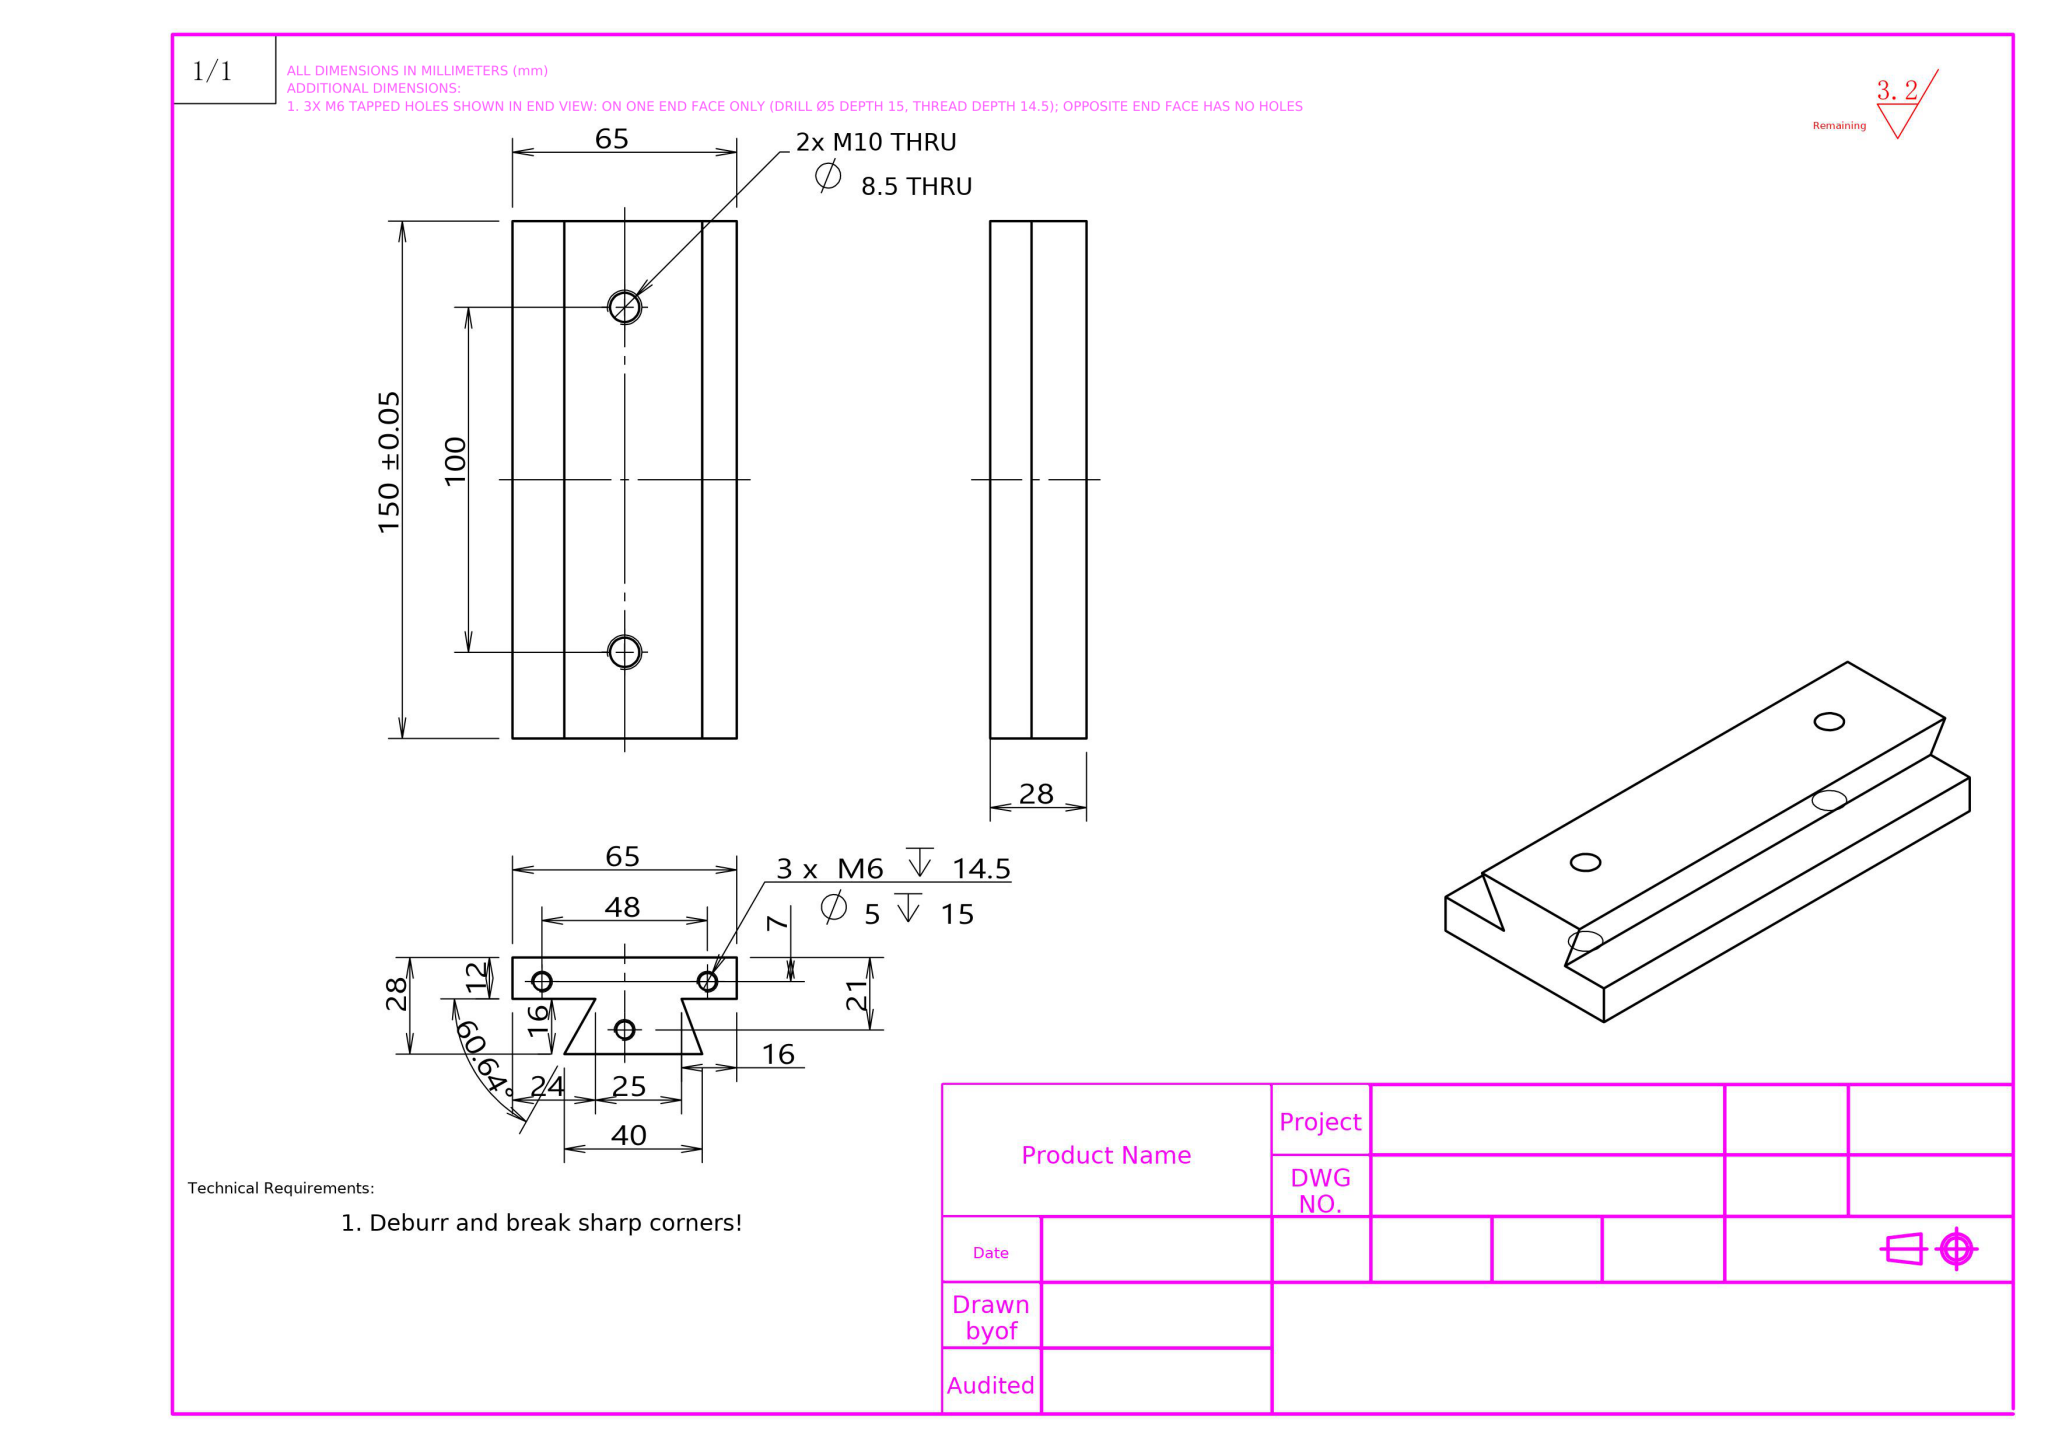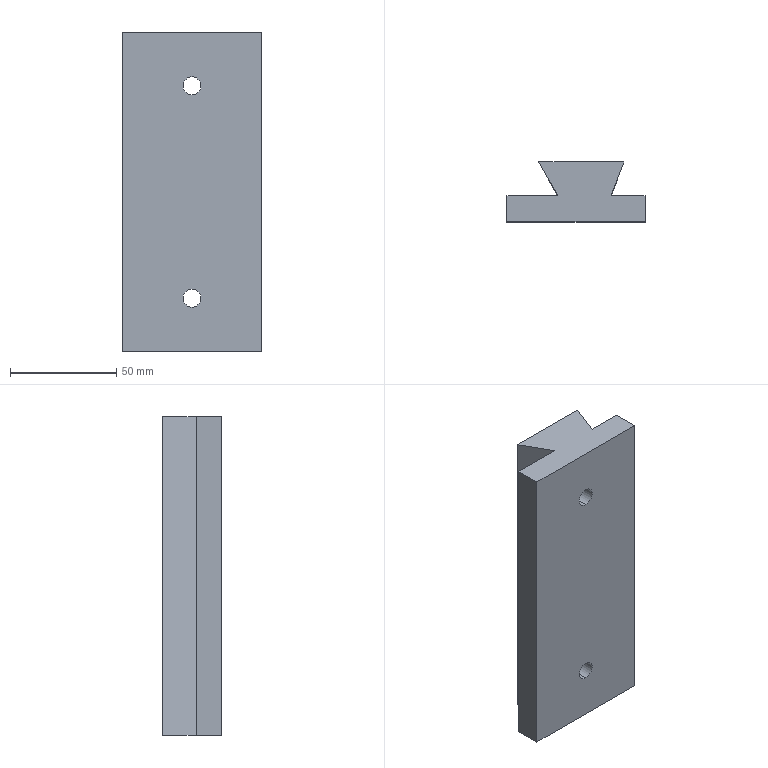Part | NX | mm | 1 solid | 26 faces | box 65 x 28 x 150 mm | volume 190909 mm3 | cylinder 10 | plane 10 | cone 6 | commonest cylinder face diameters 5 x6 8.5 x4
STEP:
#1=COLOUR_RGB('',0.7529,0.7529,0.7529);
#2=FILL_AREA_STYLE_COLOUR('',#1);
#3=FILL_AREA_STYLE('',(#2));
#4=SURFACE_STYLE_FILL_AREA(#3);
#5=SURFACE_SIDE_STYLE('',(#4));
#6=SURFACE_STYLE_USAGE(.BOTH.,#5);
#7=PRESENTATION_STYLE_ASSIGNMENT((#6));
#8=CARTESIAN_POINT('',(-21.5,1.,15.));
#9=VERTEX_POINT('',#8);
#10=CARTESIAN_POINT('',(-21.5,1.,-0.));
#11=VERTEX_POINT('',#10);
#12=CARTESIAN_POINT('',(-21.5,1.,0.));
#13=DIRECTION('',(0.,0.,-1.));
#14=VECTOR('',#13,1000.);
#15=LINE('',#12,#14);
#16=EDGE_CURVE('',#9,#11,#15,.T.);
#17=ORIENTED_EDGE('',*,*,#16,.F.);
#18=CARTESIAN_POINT('',(-26.5,1.,15.));
#19=VERTEX_POINT('',#18);
#20=CARTESIAN_POINT('',(-24.,1.,15.));
#21=DIRECTION('',(0.,0.,-1.));
#22=DIRECTION('',(-1.,0.,0.));
#23=AXIS2_PLACEMENT_3D('',#20,#21,#22);
#24=CIRCLE('',#23,2.5);
#25=EDGE_CURVE('',#19,#9,#24,.T.);
#26=ORIENTED_EDGE('',*,*,#25,.F.);
#27=CARTESIAN_POINT('',(-26.5,1.,-0.));
#28=VERTEX_POINT('',#27);
#29=CARTESIAN_POINT('',(-26.5,1.,0.));
#30=DIRECTION('',(0.,0.,-1.));
#31=VECTOR('',#30,1000.);
#32=LINE('',#29,#31);
#33=EDGE_CURVE('',#19,#28,#32,.T.);
#34=ORIENTED_EDGE('',*,*,#33,.T.);
#35=CARTESIAN_POINT('',(-24.,1.,-0.));
#36=DIRECTION('',(0.,0.,-1.));
#37=DIRECTION('',(-1.,0.,0.));
#38=AXIS2_PLACEMENT_3D('',#35,#36,#37);
#39=CIRCLE('',#38,2.5);
#40=EDGE_CURVE('',#28,#11,#39,.T.);
#41=ORIENTED_EDGE('',*,*,#40,.T.);
#42=EDGE_LOOP('',(#17,#26,#34,#41));
#43=FACE_OUTER_BOUND('',#42,.T.);
#44=CARTESIAN_POINT('',(-24.,1.,0.));
#45=DIRECTION('',(0.,0.,-1.));
#46=DIRECTION('',(-1.,0.,0.));
#47=AXIS2_PLACEMENT_3D('',#44,#45,#46);
#48=CYLINDRICAL_SURFACE('',#47,2.5);
#49=ADVANCED_FACE('',(#43),#48,.F.);
#50=STYLED_ITEM('',(#7),#49);
#51=(LENGTH_UNIT()NAMED_UNIT(*)SI_UNIT(.MILLI.,.METRE.));
#52=UNCERTAINTY_MEASURE_WITH_UNIT(LENGTH_MEASURE(0.00001),#51,'','');
#53=(NAMED_UNIT(*)PLANE_ANGLE_UNIT()SI_UNIT($,.RADIAN.));
#54=(NAMED_UNIT(*)SI_UNIT($,.STERADIAN.)SOLID_ANGLE_UNIT());
#55=(GEOMETRIC_REPRESENTATION_CONTEXT(3)GLOBAL_UNCERTAINTY_ASSIGNED_CONTEXT((#52))GLOBAL_UNIT_ASSIGNED_CONTEXT((#51,#53,#54))REPRESENTATION_CONTEXT('',''));
#56=MECHANICAL_DESIGN_GEOMETRIC_PRESENTATION_REPRESENTATION('',(#50),#55);
#57=COLOUR_RGB('',0.7529,0.7529,0.7529);
#58=FILL_AREA_STYLE_COLOUR('',#57);
#59=FILL_AREA_STYLE('',(#58));
#60=SURFACE_STYLE_FILL_AREA(#59);
#61=SURFACE_SIDE_STYLE('',(#60));
#62=SURFACE_STYLE_USAGE(.BOTH.,#61);
#63=PRESENTATION_STYLE_ASSIGNMENT((#62));
#64=CARTESIAN_POINT('',(-24.,1.,15.));
#65=DIRECTION('',(0.,0.,-1.));
#66=DIRECTION('',(-1.,0.,0.));
#67=AXIS2_PLACEMENT_3D('',#64,#65,#66);
#68=CIRCLE('',#67,2.5);
#69=EDGE_CURVE('',#9,#19,#68,.T.);
#70=ORIENTED_EDGE('',*,*,#69,.F.);
#71=ORIENTED_EDGE('',*,*,#16,.T.);
#72=CARTESIAN_POINT('',(-24.,1.,-0.));
#73=DIRECTION('',(0.,0.,-1.));
#74=DIRECTION('',(-1.,0.,0.));
#75=AXIS2_PLACEMENT_3D('',#72,#73,#74);
#76=CIRCLE('',#75,2.5);
#77=EDGE_CURVE('',#11,#28,#76,.T.);
#78=ORIENTED_EDGE('',*,*,#77,.T.);
#79=ORIENTED_EDGE('',*,*,#33,.F.);
#80=EDGE_LOOP('',(#70,#71,#78,#79));
#81=FACE_OUTER_BOUND('',#80,.T.);
#82=CARTESIAN_POINT('',(-24.,1.,0.));
#83=DIRECTION('',(0.,0.,-1.));
#84=DIRECTION('',(-1.,0.,0.));
#85=AXIS2_PLACEMENT_3D('',#82,#83,#84);
#86=CYLINDRICAL_SURFACE('',#85,2.5);
#87=ADVANCED_FACE('',(#81),#86,.F.);
#88=CARTESIAN_POINT('',(-24.,1.,16.502));
#89=VERTEX_POINT('',#88);
#90=CARTESIAN_POINT('',(-26.5,1.,15.));
#91=DIRECTION('',(-0.8572,0.,-0.515));
#92=VECTOR('',#91,1000.);
#93=LINE('',#90,#92);
#94=EDGE_CURVE('',#89,#19,#93,.T.);
#95=ORIENTED_EDGE('',*,*,#94,.F.);
#96=CARTESIAN_POINT('',(-21.5,1.,15.));
#97=DIRECTION('',(0.8572,0.,-0.515));
#98=VECTOR('',#97,1000.);
#99=LINE('',#96,#98);
#100=EDGE_CURVE('',#89,#9,#99,.T.);
#101=ORIENTED_EDGE('',*,*,#100,.T.);
#102=ORIENTED_EDGE('',*,*,#69,.T.);
#103=EDGE_LOOP('',(#95,#101,#102));
#104=FACE_OUTER_BOUND('',#103,.T.);
#105=CARTESIAN_POINT('',(-24.,1.,15.));
#106=DIRECTION('',(0.,0.,-1.));
#107=DIRECTION('',(-1.,0.,0.));
#108=AXIS2_PLACEMENT_3D('',#105,#106,#107);
#109=CONICAL_SURFACE('',#108,2.5,1.03);
#110=ADVANCED_FACE('',(#104),#109,.F.);
#111=CARTESIAN_POINT('',(2.5,15.,15.));
#112=VERTEX_POINT('',#111);
#113=CARTESIAN_POINT('',(-2.5,15.,15.));
#114=VERTEX_POINT('',#113);
#115=CARTESIAN_POINT('',(0.,15.,15.));
#116=DIRECTION('',(0.,0.,-1.));
#117=DIRECTION('',(-1.,0.,0.));
#118=AXIS2_PLACEMENT_3D('',#115,#116,#117);
#119=CIRCLE('',#118,2.5);
#120=EDGE_CURVE('',#112,#114,#119,.T.);
#121=ORIENTED_EDGE('',*,*,#120,.F.);
#122=CARTESIAN_POINT('',(2.5,15.,-0.));
#123=VERTEX_POINT('',#122);
#124=CARTESIAN_POINT('',(2.5,15.,0.));
#125=DIRECTION('',(0.,0.,-1.));
#126=VECTOR('',#125,1000.);
#127=LINE('',#124,#126);
#128=EDGE_CURVE('',#112,#123,#127,.T.);
#129=ORIENTED_EDGE('',*,*,#128,.T.);
#130=CARTESIAN_POINT('',(-2.5,15.,-0.));
#131=VERTEX_POINT('',#130);
#132=CARTESIAN_POINT('',(0.,15.,-0.));
#133=DIRECTION('',(0.,0.,-1.));
#134=DIRECTION('',(-1.,0.,0.));
#135=AXIS2_PLACEMENT_3D('',#132,#133,#134);
#136=CIRCLE('',#135,2.5);
#137=EDGE_CURVE('',#123,#131,#136,.T.);
#138=ORIENTED_EDGE('',*,*,#137,.T.);
#139=CARTESIAN_POINT('',(-2.5,15.,0.));
#140=DIRECTION('',(0.,0.,-1.));
#141=VECTOR('',#140,1000.);
#142=LINE('',#139,#141);
#143=EDGE_CURVE('',#114,#131,#142,.T.);
#144=ORIENTED_EDGE('',*,*,#143,.F.);
#145=EDGE_LOOP('',(#121,#129,#138,#144));
#146=FACE_OUTER_BOUND('',#145,.T.);
#147=CARTESIAN_POINT('',(0.,15.,0.));
#148=DIRECTION('',(0.,0.,-1.));
#149=DIRECTION('',(-1.,0.,0.));
#150=AXIS2_PLACEMENT_3D('',#147,#148,#149);
#151=CYLINDRICAL_SURFACE('',#150,2.5);
#152=ADVANCED_FACE('',(#146),#151,.F.);
#153=CARTESIAN_POINT('',(0.,15.,16.502));
#154=VERTEX_POINT('',#153);
#155=CARTESIAN_POINT('',(-2.5,15.,15.));
#156=DIRECTION('',(-0.8572,0.,-0.515));
#157=VECTOR('',#156,1000.);
#158=LINE('',#155,#157);
#159=EDGE_CURVE('',#154,#114,#158,.T.);
#160=ORIENTED_EDGE('',*,*,#159,.F.);
#161=CARTESIAN_POINT('',(2.5,15.,15.));
#162=DIRECTION('',(0.8572,0.,-0.515));
#163=VECTOR('',#162,1000.);
#164=LINE('',#161,#163);
#165=EDGE_CURVE('',#154,#112,#164,.T.);
#166=ORIENTED_EDGE('',*,*,#165,.T.);
#167=ORIENTED_EDGE('',*,*,#120,.T.);
#168=EDGE_LOOP('',(#160,#166,#167));
#169=FACE_OUTER_BOUND('',#168,.T.);
#170=CARTESIAN_POINT('',(0.,15.,15.));
#171=DIRECTION('',(0.,0.,-1.));
#172=DIRECTION('',(-1.,0.,0.));
#173=AXIS2_PLACEMENT_3D('',#170,#171,#172);
#174=CONICAL_SURFACE('',#173,2.5,1.03);
#175=ADVANCED_FACE('',(#169),#174,.F.);
#176=CARTESIAN_POINT('',(26.5,1.,15.));
#177=VERTEX_POINT('',#176);
#178=CARTESIAN_POINT('',(21.5,1.,15.));
#179=VERTEX_POINT('',#178);
#180=CARTESIAN_POINT('',(24.,1.,15.));
#181=DIRECTION('',(0.,0.,-1.));
#182=DIRECTION('',(-1.,0.,0.));
#183=AXIS2_PLACEMENT_3D('',#180,#181,#182);
#184=CIRCLE('',#183,2.5);
#185=EDGE_CURVE('',#177,#179,#184,.T.);
#186=ORIENTED_EDGE('',*,*,#185,.F.);
#187=CARTESIAN_POINT('',(26.5,1.,-0.));
#188=VERTEX_POINT('',#187);
#189=CARTESIAN_POINT('',(26.5,1.,0.));
#190=DIRECTION('',(0.,0.,-1.));
#191=VECTOR('',#190,1000.);
#192=LINE('',#189,#191);
#193=EDGE_CURVE('',#177,#188,#192,.T.);
#194=ORIENTED_EDGE('',*,*,#193,.T.);
#195=CARTESIAN_POINT('',(21.5,1.,-0.));
#196=VERTEX_POINT('',#195);
#197=CARTESIAN_POINT('',(24.,1.,-0.));
#198=DIRECTION('',(0.,0.,-1.));
#199=DIRECTION('',(-1.,0.,0.));
#200=AXIS2_PLACEMENT_3D('',#197,#198,#199);
#201=CIRCLE('',#200,2.5);
#202=EDGE_CURVE('',#188,#196,#201,.T.);
#203=ORIENTED_EDGE('',*,*,#202,.T.);
#204=CARTESIAN_POINT('',(21.5,1.,0.));
#205=DIRECTION('',(0.,0.,-1.));
#206=VECTOR('',#205,1000.);
#207=LINE('',#204,#206);
#208=EDGE_CURVE('',#179,#196,#207,.T.);
#209=ORIENTED_EDGE('',*,*,#208,.F.);
#210=EDGE_LOOP('',(#186,#194,#203,#209));
#211=FACE_OUTER_BOUND('',#210,.T.);
#212=CARTESIAN_POINT('',(24.,1.,0.));
#213=DIRECTION('',(0.,0.,-1.));
#214=DIRECTION('',(-1.,0.,0.));
#215=AXIS2_PLACEMENT_3D('',#212,#213,#214);
#216=CYLINDRICAL_SURFACE('',#215,2.5);
#217=ADVANCED_FACE('',(#211),#216,.F.);
#218=CARTESIAN_POINT('',(24.,1.,16.502));
#219=VERTEX_POINT('',#218);
#220=CARTESIAN_POINT('',(21.5,1.,15.));
#221=DIRECTION('',(-0.8572,0.,-0.515));
#222=VECTOR('',#221,1000.);
#223=LINE('',#220,#222);
#224=EDGE_CURVE('',#219,#179,#223,.T.);
#225=ORIENTED_EDGE('',*,*,#224,.F.);
#226=CARTESIAN_POINT('',(26.5,1.,15.));
#227=DIRECTION('',(0.8572,0.,-0.515));
#228=VECTOR('',#227,1000.);
#229=LINE('',#226,#228);
#230=EDGE_CURVE('',#219,#177,#229,.T.);
#231=ORIENTED_EDGE('',*,*,#230,.T.);
#232=ORIENTED_EDGE('',*,*,#185,.T.);
#233=EDGE_LOOP('',(#225,#231,#232));
#234=FACE_OUTER_BOUND('',#233,.T.);
#235=CARTESIAN_POINT('',(24.,1.,15.));
#236=DIRECTION('',(0.,0.,-1.));
#237=DIRECTION('',(-1.,0.,0.));
#238=AXIS2_PLACEMENT_3D('',#235,#236,#237);
#239=CONICAL_SURFACE('',#238,2.5,1.03);
#240=ADVANCED_FACE('',(#234),#239,.F.);
#241=CARTESIAN_POINT('',(0.,22.,129.25));
#242=VERTEX_POINT('',#241);
#243=CARTESIAN_POINT('',(0.,22.,120.75));
#244=VERTEX_POINT('',#243);
#245=CARTESIAN_POINT('',(0.,22.,125.));
#246=DIRECTION('',(0.,-1.,0.));
#247=DIRECTION('',(0.,0.,-1.));
#248=AXIS2_PLACEMENT_3D('',#245,#246,#247);
#249=CIRCLE('',#248,4.25);
#250=EDGE_CURVE('',#242,#244,#249,.T.);
#251=ORIENTED_EDGE('',*,*,#250,.F.);
#252=CARTESIAN_POINT('',(0.,-6.,129.25));
#253=VERTEX_POINT('',#252);
#254=CARTESIAN_POINT('',(0.,-6.,129.25));
#255=DIRECTION('',(0.,-1.,0.));
#256=VECTOR('',#255,1000.);
#257=LINE('',#254,#256);
#258=EDGE_CURVE('',#242,#253,#257,.T.);
#259=ORIENTED_EDGE('',*,*,#258,.T.);
#260=CARTESIAN_POINT('',(0.,-6.,120.75));
#261=VERTEX_POINT('',#260);
#262=CARTESIAN_POINT('',(0.,-6.,125.));
#263=DIRECTION('',(0.,-1.,0.));
#264=DIRECTION('',(0.,0.,-1.));
#265=AXIS2_PLACEMENT_3D('',#262,#263,#264);
#266=CIRCLE('',#265,4.25);
#267=EDGE_CURVE('',#253,#261,#266,.T.);
#268=ORIENTED_EDGE('',*,*,#267,.T.);
#269=CARTESIAN_POINT('',(0.,-6.,120.75));
#270=DIRECTION('',(0.,-1.,0.));
#271=VECTOR('',#270,1000.);
#272=LINE('',#269,#271);
#273=EDGE_CURVE('',#244,#261,#272,.T.);
#274=ORIENTED_EDGE('',*,*,#273,.F.);
#275=EDGE_LOOP('',(#251,#259,#268,#274));
#276=FACE_OUTER_BOUND('',#275,.T.);
#277=CARTESIAN_POINT('',(0.,-6.,125.));
#278=DIRECTION('',(0.,-1.,0.));
#279=DIRECTION('',(0.,0.,-1.));
#280=AXIS2_PLACEMENT_3D('',#277,#278,#279);
#281=CYLINDRICAL_SURFACE('',#280,4.25);
#282=ADVANCED_FACE('',(#276),#281,.F.);
#283=CARTESIAN_POINT('',(0.,22.,29.25));
#284=VERTEX_POINT('',#283);
#285=CARTESIAN_POINT('',(0.,22.,20.75));
#286=VERTEX_POINT('',#285);
#287=CARTESIAN_POINT('',(0.,22.,25.));
#288=DIRECTION('',(0.,-1.,0.));
#289=DIRECTION('',(0.,0.,-1.));
#290=AXIS2_PLACEMENT_3D('',#287,#288,#289);
#291=CIRCLE('',#290,4.25);
#292=EDGE_CURVE('',#284,#286,#291,.T.);
#293=ORIENTED_EDGE('',*,*,#292,.F.);
#294=CARTESIAN_POINT('',(0.,-6.,29.25));
#295=VERTEX_POINT('',#294);
#296=CARTESIAN_POINT('',(0.,-6.,29.25));
#297=DIRECTION('',(0.,-1.,0.));
#298=VECTOR('',#297,1000.);
#299=LINE('',#296,#298);
#300=EDGE_CURVE('',#284,#295,#299,.T.);
#301=ORIENTED_EDGE('',*,*,#300,.T.);
#302=CARTESIAN_POINT('',(0.,-6.,20.75));
#303=VERTEX_POINT('',#302);
#304=CARTESIAN_POINT('',(0.,-6.,25.));
#305=DIRECTION('',(0.,-1.,0.));
#306=DIRECTION('',(0.,0.,-1.));
#307=AXIS2_PLACEMENT_3D('',#304,#305,#306);
#308=CIRCLE('',#307,4.25);
#309=EDGE_CURVE('',#295,#303,#308,.T.);
#310=ORIENTED_EDGE('',*,*,#309,.T.);
#311=CARTESIAN_POINT('',(0.,-6.,20.75));
#312=DIRECTION('',(0.,-1.,0.));
#313=VECTOR('',#312,1000.);
#314=LINE('',#311,#313);
#315=EDGE_CURVE('',#286,#303,#314,.T.);
#316=ORIENTED_EDGE('',*,*,#315,.F.);
#317=EDGE_LOOP('',(#293,#301,#310,#316));
#318=FACE_OUTER_BOUND('',#317,.T.);
#319=CARTESIAN_POINT('',(0.,-6.,25.));
#320=DIRECTION('',(0.,-1.,0.));
#321=DIRECTION('',(0.,0.,-1.));
#322=AXIS2_PLACEMENT_3D('',#319,#320,#321);
#323=CYLINDRICAL_SURFACE('',#322,4.25);
#324=ADVANCED_FACE('',(#318),#323,.F.);
#325=CARTESIAN_POINT('',(32.5,-6.,0.));
#326=VERTEX_POINT('',#325);
#327=CARTESIAN_POINT('',(32.5,6.,0.));
#328=VERTEX_POINT('',#327);
#329=CARTESIAN_POINT('',(32.5,6.,0.));
#330=DIRECTION('',(0.,1.,0.));
#331=VECTOR('',#330,1000.);
#332=LINE('',#329,#331);
#333=EDGE_CURVE('',#326,#328,#332,.T.);
#334=ORIENTED_EDGE('',*,*,#333,.T.);
#335=CARTESIAN_POINT('',(32.5,6.,150.));
#336=VERTEX_POINT('',#335);
#337=CARTESIAN_POINT('',(32.5,6.,150.));
#338=DIRECTION('',(0.,0.,-1.));
#339=VECTOR('',#338,1000.);
#340=LINE('',#337,#339);
#341=EDGE_CURVE('',#336,#328,#340,.T.);
#342=ORIENTED_EDGE('',*,*,#341,.F.);
#343=CARTESIAN_POINT('',(32.5,-6.,150.));
#344=VERTEX_POINT('',#343);
#345=CARTESIAN_POINT('',(32.5,6.,150.));
#346=DIRECTION('',(0.,1.,0.));
#347=VECTOR('',#346,1000.);
#348=LINE('',#345,#347);
#349=EDGE_CURVE('',#344,#336,#348,.T.);
#350=ORIENTED_EDGE('',*,*,#349,.F.);
#351=CARTESIAN_POINT('',(32.5,-6.,150.));
#352=DIRECTION('',(0.,0.,-1.));
#353=VECTOR('',#352,1000.);
#354=LINE('',#351,#353);
#355=EDGE_CURVE('',#344,#326,#354,.T.);
#356=ORIENTED_EDGE('',*,*,#355,.T.);
#357=EDGE_LOOP('',(#334,#342,#350,#356));
#358=FACE_OUTER_BOUND('',#357,.T.);
#359=CARTESIAN_POINT('',(32.5,6.,150.));
#360=DIRECTION('',(-1.,0.,0.));
#361=DIRECTION('',(0.,0.,1.));
#362=AXIS2_PLACEMENT_3D('',#359,#360,#361);
#363=PLANE('',#362);
#364=ADVANCED_FACE('',(#358),#363,.F.);
#365=CARTESIAN_POINT('',(16.5,6.,0.));
#366=VERTEX_POINT('',#365);
#367=CARTESIAN_POINT('',(16.5,6.,0.));
#368=DIRECTION('',(-1.,0.,0.));
#369=VECTOR('',#368,1000.);
#370=LINE('',#367,#369);
#371=EDGE_CURVE('',#328,#366,#370,.T.);
#372=ORIENTED_EDGE('',*,*,#371,.T.);
#373=CARTESIAN_POINT('',(16.5,6.,150.));
#374=VERTEX_POINT('',#373);
#375=CARTESIAN_POINT('',(16.5,6.,150.));
#376=DIRECTION('',(0.,0.,-1.));
#377=VECTOR('',#376,1000.);
#378=LINE('',#375,#377);
#379=EDGE_CURVE('',#374,#366,#378,.T.);
#380=ORIENTED_EDGE('',*,*,#379,.F.);
#381=CARTESIAN_POINT('',(16.5,6.,150.));
#382=DIRECTION('',(-1.,0.,0.));
#383=VECTOR('',#382,1000.);
#384=LINE('',#381,#383);
#385=EDGE_CURVE('',#336,#374,#384,.T.);
#386=ORIENTED_EDGE('',*,*,#385,.F.);
#387=ORIENTED_EDGE('',*,*,#341,.T.);
#388=EDGE_LOOP('',(#372,#380,#386,#387));
#389=FACE_OUTER_BOUND('',#388,.T.);
#390=CARTESIAN_POINT('',(16.5,6.,150.));
#391=DIRECTION('',(0.,-1.,0.));
#392=DIRECTION('',(0.,0.,-1.));
#393=AXIS2_PLACEMENT_3D('',#390,#391,#392);
#394=PLANE('',#393);
#395=ADVANCED_FACE('',(#389),#394,.F.);
#396=CARTESIAN_POINT('',(22.5,22.,0.));
#397=VERTEX_POINT('',#396);
#398=CARTESIAN_POINT('',(22.5,22.,0.));
#399=DIRECTION('',(0.3511,0.9363,0.));
#400=VECTOR('',#399,1000.);
#401=LINE('',#398,#400);
#402=EDGE_CURVE('',#366,#397,#401,.T.);
#403=ORIENTED_EDGE('',*,*,#402,.T.);
#404=CARTESIAN_POINT('',(22.5,22.,150.));
#405=VERTEX_POINT('',#404);
#406=CARTESIAN_POINT('',(22.5,22.,150.));
#407=DIRECTION('',(0.,0.,-1.));
#408=VECTOR('',#407,1000.);
#409=LINE('',#406,#408);
#410=EDGE_CURVE('',#405,#397,#409,.T.);
#411=ORIENTED_EDGE('',*,*,#410,.F.);
#412=CARTESIAN_POINT('',(22.5,22.,150.));
#413=DIRECTION('',(0.3511,0.9363,0.));
#414=VECTOR('',#413,1000.);
#415=LINE('',#412,#414);
#416=EDGE_CURVE('',#374,#405,#415,.T.);
#417=ORIENTED_EDGE('',*,*,#416,.F.);
#418=ORIENTED_EDGE('',*,*,#379,.T.);
#419=EDGE_LOOP('',(#403,#411,#417,#418));
#420=FACE_OUTER_BOUND('',#419,.T.);
#421=CARTESIAN_POINT('',(22.5,22.,150.));
#422=DIRECTION('',(-0.9363,0.3511,0.));
#423=DIRECTION('',(-0.3511,-0.9363,0.));
#424=AXIS2_PLACEMENT_3D('',#421,#422,#423);
#425=PLANE('',#424);
#426=ADVANCED_FACE('',(#420),#425,.F.);
#427=CARTESIAN_POINT('',(0.,22.,125.));
#428=DIRECTION('',(0.,-1.,0.));
#429=DIRECTION('',(0.,0.,-1.));
#430=AXIS2_PLACEMENT_3D('',#427,#428,#429);
#431=CIRCLE('',#430,4.25);
#432=EDGE_CURVE('',#244,#242,#431,.T.);
#433=ORIENTED_EDGE('',*,*,#432,.T.);
#434=ORIENTED_EDGE('',*,*,#250,.T.);
#435=EDGE_LOOP('',(#433,#434));
#436=FACE_BOUND('',#435,.T.);
#437=CARTESIAN_POINT('',(0.,22.,25.));
#438=DIRECTION('',(0.,-1.,0.));
#439=DIRECTION('',(0.,0.,-1.));
#440=AXIS2_PLACEMENT_3D('',#437,#438,#439);
#441=CIRCLE('',#440,4.25);
#442=EDGE_CURVE('',#286,#284,#441,.T.);
#443=ORIENTED_EDGE('',*,*,#442,.T.);
#444=ORIENTED_EDGE('',*,*,#292,.T.);
#445=EDGE_LOOP('',(#443,#444));
#446=FACE_BOUND('',#445,.T.);
#447=CARTESIAN_POINT('',(-17.5,22.,0.));
#448=VERTEX_POINT('',#447);
#449=CARTESIAN_POINT('',(-17.5,22.,0.));
#450=DIRECTION('',(-1.,0.,0.));
#451=VECTOR('',#450,1000.);
#452=LINE('',#449,#451);
#453=EDGE_CURVE('',#397,#448,#452,.T.);
#454=ORIENTED_EDGE('',*,*,#453,.T.);
#455=CARTESIAN_POINT('',(-17.5,22.,150.));
#456=VERTEX_POINT('',#455);
#457=CARTESIAN_POINT('',(-17.5,22.,150.));
#458=DIRECTION('',(0.,0.,-1.));
#459=VECTOR('',#458,1000.);
#460=LINE('',#457,#459);
#461=EDGE_CURVE('',#456,#448,#460,.T.);
#462=ORIENTED_EDGE('',*,*,#461,.F.);
#463=CARTESIAN_POINT('',(-17.5,22.,150.));
#464=DIRECTION('',(-1.,0.,0.));
#465=VECTOR('',#464,1000.);
#466=LINE('',#463,#465);
#467=EDGE_CURVE('',#405,#456,#466,.T.);
#468=ORIENTED_EDGE('',*,*,#467,.F.);
#469=ORIENTED_EDGE('',*,*,#410,.T.);
#470=EDGE_LOOP('',(#454,#462,#468,#469));
#471=FACE_OUTER_BOUND('',#470,.T.);
#472=CARTESIAN_POINT('',(-17.5,22.,150.));
#473=DIRECTION('',(0.,-1.,0.));
#474=DIRECTION('',(0.,0.,-1.));
#475=AXIS2_PLACEMENT_3D('',#472,#473,#474);
#476=PLANE('',#475);
#477=ADVANCED_FACE('',(#436,#446,#471),#476,.F.);
#478=CARTESIAN_POINT('',(-8.5,6.,0.));
#479=VERTEX_POINT('',#478);
#480=CARTESIAN_POINT('',(-8.5,6.,0.));
#481=DIRECTION('',(0.4903,-0.8716,0.));
#482=VECTOR('',#481,1000.);
#483=LINE('',#480,#482);
#484=EDGE_CURVE('',#448,#479,#483,.T.);
#485=ORIENTED_EDGE('',*,*,#484,.T.);
#486=CARTESIAN_POINT('',(-8.5,6.,150.));
#487=VERTEX_POINT('',#486);
#488=CARTESIAN_POINT('',(-8.5,6.,150.));
#489=DIRECTION('',(0.,0.,-1.));
#490=VECTOR('',#489,1000.);
#491=LINE('',#488,#490);
#492=EDGE_CURVE('',#487,#479,#491,.T.);
#493=ORIENTED_EDGE('',*,*,#492,.F.);
#494=CARTESIAN_POINT('',(-8.5,6.,150.));
#495=DIRECTION('',(0.4903,-0.8716,0.));
#496=VECTOR('',#495,1000.);
#497=LINE('',#494,#496);
#498=EDGE_CURVE('',#456,#487,#497,.T.);
#499=ORIENTED_EDGE('',*,*,#498,.F.);
#500=ORIENTED_EDGE('',*,*,#461,.T.);
#501=EDGE_LOOP('',(#485,#493,#499,#500));
#502=FACE_OUTER_BOUND('',#501,.T.);
#503=CARTESIAN_POINT('',(-8.5,6.,150.));
#504=DIRECTION('',(0.8716,0.4903,0.));
#505=DIRECTION('',(-0.4903,0.8716,0.));
#506=AXIS2_PLACEMENT_3D('',#503,#504,#505);
#507=PLANE('',#506);
#508=ADVANCED_FACE('',(#502),#507,.F.);
#509=CARTESIAN_POINT('',(-32.5,6.,0.));
#510=VERTEX_POINT('',#509);
#511=CARTESIAN_POINT('',(-32.5,6.,0.));
#512=DIRECTION('',(-1.,0.,0.));
#513=VECTOR('',#512,1000.);
#514=LINE('',#511,#513);
#515=EDGE_CURVE('',#479,#510,#514,.T.);
#516=ORIENTED_EDGE('',*,*,#515,.T.);
#517=CARTESIAN_POINT('',(-32.5,6.,150.));
#518=VERTEX_POINT('',#517);
#519=CARTESIAN_POINT('',(-32.5,6.,150.));
#520=DIRECTION('',(0.,0.,-1.));
#521=VECTOR('',#520,1000.);
#522=LINE('',#519,#521);
#523=EDGE_CURVE('',#518,#510,#522,.T.);
#524=ORIENTED_EDGE('',*,*,#523,.F.);
#525=CARTESIAN_POINT('',(-32.5,6.,150.));
#526=DIRECTION('',(-1.,0.,0.));
#527=VECTOR('',#526,1000.);
#528=LINE('',#525,#527);
#529=EDGE_CURVE('',#487,#518,#528,.T.);
#530=ORIENTED_EDGE('',*,*,#529,.F.);
#531=ORIENTED_EDGE('',*,*,#492,.T.);
#532=EDGE_LOOP('',(#516,#524,#530,#531));
#533=FACE_OUTER_BOUND('',#532,.T.);
#534=CARTESIAN_POINT('',(-32.5,6.,150.));
#535=DIRECTION('',(0.,-1.,0.));
#536=DIRECTION('',(0.,0.,-1.));
#537=AXIS2_PLACEMENT_3D('',#534,#535,#536);
#538=PLANE('',#537);
#539=ADVANCED_FACE('',(#533),#538,.F.);
#540=CARTESIAN_POINT('',(-32.5,-6.,0.));
#541=VERTEX_POINT('',#540);
#542=CARTESIAN_POINT('',(-32.5,6.,0.));
#543=DIRECTION('',(0.,-1.,0.));
#544=VECTOR('',#543,1000.);
#545=LINE('',#542,#544);
#546=EDGE_CURVE('',#510,#541,#545,.T.);
#547=ORIENTED_EDGE('',*,*,#546,.T.);
#548=CARTESIAN_POINT('',(-32.5,-6.,150.));
#549=VERTEX_POINT('',#548);
#550=CARTESIAN_POINT('',(-32.5,-6.,150.));
#551=DIRECTION('',(0.,0.,-1.));
#552=VECTOR('',#551,1000.);
#553=LINE('',#550,#552);
#554=EDGE_CURVE('',#549,#541,#553,.T.);
#555=ORIENTED_EDGE('',*,*,#554,.F.);
#556=CARTESIAN_POINT('',(-32.5,6.,150.));
#557=DIRECTION('',(0.,-1.,0.));
#558=VECTOR('',#557,1000.);
#559=LINE('',#556,#558);
#560=EDGE_CURVE('',#518,#549,#559,.T.);
#561=ORIENTED_EDGE('',*,*,#560,.F.);
#562=ORIENTED_EDGE('',*,*,#523,.T.);
#563=EDGE_LOOP('',(#547,#555,#561,#562));
#564=FACE_OUTER_BOUND('',#563,.T.);
#565=CARTESIAN_POINT('',(-32.5,6.,150.));
#566=DIRECTION('',(1.,0.,0.));
#567=DIRECTION('',(0.,0.,-1.));
#568=AXIS2_PLACEMENT_3D('',#565,#566,#567);
#569=PLANE('',#568);
#570=ADVANCED_FACE('',(#564),#569,.F.);
#571=CARTESIAN_POINT('',(0.,-6.,125.));
#572=DIRECTION('',(0.,-1.,0.));
#573=DIRECTION('',(0.,0.,-1.));
#574=AXIS2_PLACEMENT_3D('',#571,#572,#573);
#575=CIRCLE('',#574,4.25);
#576=EDGE_CURVE('',#261,#253,#575,.T.);
#577=ORIENTED_EDGE('',*,*,#576,.F.);
#578=ORIENTED_EDGE('',*,*,#267,.F.);
#579=EDGE_LOOP('',(#577,#578));
#580=FACE_BOUND('',#579,.T.);
#581=CARTESIAN_POINT('',(0.,-6.,25.));
#582=DIRECTION('',(0.,-1.,0.));
#583=DIRECTION('',(0.,0.,-1.));
#584=AXIS2_PLACEMENT_3D('',#581,#582,#583);
#585=CIRCLE('',#584,4.25);
#586=EDGE_CURVE('',#303,#295,#585,.T.);
#587=ORIENTED_EDGE('',*,*,#586,.F.);
#588=ORIENTED_EDGE('',*,*,#309,.F.);
#589=EDGE_LOOP('',(#587,#588));
#590=FACE_BOUND('',#589,.T.);
#591=CARTESIAN_POINT('',(-32.5,-6.,0.));
#592=DIRECTION('',(1.,0.,0.));
#593=VECTOR('',#592,1000.);
#594=LINE('',#591,#593);
#595=EDGE_CURVE('',#541,#326,#594,.T.);
#596=ORIENTED_EDGE('',*,*,#595,.T.);
#597=ORIENTED_EDGE('',*,*,#355,.F.);
#598=CARTESIAN_POINT('',(-32.5,-6.,150.));
#599=DIRECTION('',(1.,0.,0.));
#600=VECTOR('',#599,1000.);
#601=LINE('',#598,#600);
#602=EDGE_CURVE('',#549,#344,#601,.T.);
#603=ORIENTED_EDGE('',*,*,#602,.F.);
#604=ORIENTED_EDGE('',*,*,#554,.T.);
#605=EDGE_LOOP('',(#596,#597,#603,#604));
#606=FACE_OUTER_BOUND('',#605,.T.);
#607=CARTESIAN_POINT('',(-32.5,-6.,150.));
#608=DIRECTION('',(0.,1.,0.));
#609=DIRECTION('',(0.,0.,1.));
#610=AXIS2_PLACEMENT_3D('',#607,#608,#609);
#611=PLANE('',#610);
#612=ADVANCED_FACE('',(#580,#590,#606),#611,.F.);
#613=ORIENTED_EDGE('',*,*,#349,.T.);
#614=ORIENTED_EDGE('',*,*,#385,.T.);
#615=ORIENTED_EDGE('',*,*,#416,.T.);
#616=ORIENTED_EDGE('',*,*,#467,.T.);
#617=ORIENTED_EDGE('',*,*,#498,.T.);
#618=ORIENTED_EDGE('',*,*,#529,.T.);
#619=ORIENTED_EDGE('',*,*,#560,.T.);
#620=ORIENTED_EDGE('',*,*,#602,.T.);
#621=EDGE_LOOP('',(#613,#614,#615,#616,#617,#618,#619,#620));
#622=FACE_OUTER_BOUND('',#621,.T.);
#623=CARTESIAN_POINT('',(0.,0.,150.));
#624=DIRECTION('',(0.,0.,1.));
#625=DIRECTION('',(1.,0.,0.));
#626=AXIS2_PLACEMENT_3D('',#623,#624,#625);
#627=PLANE('',#626);
#628=ADVANCED_FACE('',(#622),#627,.T.);
#629=ORIENTED_EDGE('',*,*,#40,.F.);
#630=ORIENTED_EDGE('',*,*,#77,.F.);
#631=EDGE_LOOP('',(#629,#630));
#632=FACE_BOUND('',#631,.T.);
#633=CARTESIAN_POINT('',(0.,15.,-0.));
#634=DIRECTION('',(0.,0.,-1.));
#635=DIRECTION('',(-1.,0.,0.));
#636=AXIS2_PLACEMENT_3D('',#633,#634,#635);
#637=CIRCLE('',#636,2.5);
#638=EDGE_CURVE('',#131,#123,#637,.T.);
#639=ORIENTED_EDGE('',*,*,#638,.F.);
#640=ORIENTED_EDGE('',*,*,#137,.F.);
#641=EDGE_LOOP('',(#639,#640));
#642=FACE_BOUND('',#641,.T.);
#643=CARTESIAN_POINT('',(24.,1.,-0.));
#644=DIRECTION('',(0.,0.,-1.));
#645=DIRECTION('',(-1.,0.,0.));
#646=AXIS2_PLACEMENT_3D('',#643,#644,#645);
#647=CIRCLE('',#646,2.5);
#648=EDGE_CURVE('',#196,#188,#647,.T.);
#649=ORIENTED_EDGE('',*,*,#648,.F.);
#650=ORIENTED_EDGE('',*,*,#202,.F.);
#651=EDGE_LOOP('',(#649,#650));
#652=FACE_BOUND('',#651,.T.);
#653=ORIENTED_EDGE('',*,*,#333,.F.);
#654=ORIENTED_EDGE('',*,*,#595,.F.);
#655=ORIENTED_EDGE('',*,*,#546,.F.);
#656=ORIENTED_EDGE('',*,*,#515,.F.);
#657=ORIENTED_EDGE('',*,*,#484,.F.);
#658=ORIENTED_EDGE('',*,*,#453,.F.);
#659=ORIENTED_EDGE('',*,*,#402,.F.);
#660=ORIENTED_EDGE('',*,*,#371,.F.);
#661=EDGE_LOOP('',(#653,#654,#655,#656,#657,#658,#659,#660));
#662=FACE_OUTER_BOUND('',#661,.T.);
#663=CARTESIAN_POINT('',(0.,0.,0.));
#664=DIRECTION('',(0.,0.,1.));
#665=DIRECTION('',(1.,0.,0.));
#666=AXIS2_PLACEMENT_3D('',#663,#664,#665);
#667=PLANE('',#666);
#668=ADVANCED_FACE('',(#632,#642,#652,#662),#667,.F.);
#669=ORIENTED_EDGE('',*,*,#300,.F.);
#670=ORIENTED_EDGE('',*,*,#442,.F.);
#671=ORIENTED_EDGE('',*,*,#315,.T.);
#672=ORIENTED_EDGE('',*,*,#586,.T.);
#673=EDGE_LOOP('',(#669,#670,#671,#672));
#674=FACE_OUTER_BOUND('',#673,.T.);
#675=CARTESIAN_POINT('',(0.,-6.,25.));
#676=DIRECTION('',(0.,-1.,0.));
#677=DIRECTION('',(0.,0.,-1.));
#678=AXIS2_PLACEMENT_3D('',#675,#676,#677);
#679=CYLINDRICAL_SURFACE('',#678,4.25);
#680=ADVANCED_FACE('',(#674),#679,.F.);
#681=ORIENTED_EDGE('',*,*,#258,.F.);
#682=ORIENTED_EDGE('',*,*,#432,.F.);
#683=ORIENTED_EDGE('',*,*,#273,.T.);
#684=ORIENTED_EDGE('',*,*,#576,.T.);
#685=EDGE_LOOP('',(#681,#682,#683,#684));
#686=FACE_OUTER_BOUND('',#685,.T.);
#687=CARTESIAN_POINT('',(0.,-6.,125.));
#688=DIRECTION('',(0.,-1.,0.));
#689=DIRECTION('',(0.,0.,-1.));
#690=AXIS2_PLACEMENT_3D('',#687,#688,#689);
#691=CYLINDRICAL_SURFACE('',#690,4.25);
#692=ADVANCED_FACE('',(#686),#691,.F.);
#693=ORIENTED_EDGE('',*,*,#230,.F.);
#694=ORIENTED_EDGE('',*,*,#224,.T.);
#695=CARTESIAN_POINT('',(24.,1.,15.));
#696=DIRECTION('',(0.,0.,-1.));
#697=DIRECTION('',(-1.,0.,0.));
#698=AXIS2_PLACEMENT_3D('',#695,#696,#697);
#699=CIRCLE('',#698,2.5);
#700=EDGE_CURVE('',#179,#177,#699,.T.);
#701=ORIENTED_EDGE('',*,*,#700,.T.);
#702=EDGE_LOOP('',(#693,#694,#701));
#703=FACE_OUTER_BOUND('',#702,.T.);
#704=CARTESIAN_POINT('',(24.,1.,15.));
#705=DIRECTION('',(0.,0.,-1.));
#706=DIRECTION('',(-1.,0.,0.));
#707=AXIS2_PLACEMENT_3D('',#704,#705,#706);
#708=CONICAL_SURFACE('',#707,2.5,1.03);
#709=ADVANCED_FACE('',(#703),#708,.F.);
#710=ORIENTED_EDGE('',*,*,#193,.F.);
#711=ORIENTED_EDGE('',*,*,#700,.F.);
#712=ORIENTED_EDGE('',*,*,#208,.T.);
#713=ORIENTED_EDGE('',*,*,#648,.T.);
#714=EDGE_LOOP('',(#710,#711,#712,#713));
#715=FACE_OUTER_BOUND('',#714,.T.);
#716=CARTESIAN_POINT('',(24.,1.,0.));
#717=DIRECTION('',(0.,0.,-1.));
#718=DIRECTION('',(-1.,0.,0.));
#719=AXIS2_PLACEMENT_3D('',#716,#717,#718);
#720=CYLINDRICAL_SURFACE('',#719,2.5);
#721=ADVANCED_FACE('',(#715),#720,.F.);
#722=ORIENTED_EDGE('',*,*,#165,.F.);
#723=ORIENTED_EDGE('',*,*,#159,.T.);
#724=CARTESIAN_POINT('',(0.,15.,15.));
#725=DIRECTION('',(0.,0.,-1.));
#726=DIRECTION('',(-1.,0.,0.));
#727=AXIS2_PLACEMENT_3D('',#724,#725,#726);
#728=CIRCLE('',#727,2.5);
#729=EDGE_CURVE('',#114,#112,#728,.T.);
#730=ORIENTED_EDGE('',*,*,#729,.T.);
#731=EDGE_LOOP('',(#722,#723,#730));
#732=FACE_OUTER_BOUND('',#731,.T.);
#733=CARTESIAN_POINT('',(0.,15.,15.));
#734=DIRECTION('',(0.,0.,-1.));
#735=DIRECTION('',(-1.,0.,0.));
#736=AXIS2_PLACEMENT_3D('',#733,#734,#735);
#737=CONICAL_SURFACE('',#736,2.5,1.03);
#738=ADVANCED_FACE('',(#732),#737,.F.);
#739=ORIENTED_EDGE('',*,*,#128,.F.);
#740=ORIENTED_EDGE('',*,*,#729,.F.);
#741=ORIENTED_EDGE('',*,*,#143,.T.);
#742=ORIENTED_EDGE('',*,*,#638,.T.);
#743=EDGE_LOOP('',(#739,#740,#741,#742));
#744=FACE_OUTER_BOUND('',#743,.T.);
#745=CARTESIAN_POINT('',(0.,15.,0.));
#746=DIRECTION('',(0.,0.,-1.));
#747=DIRECTION('',(-1.,0.,0.));
#748=AXIS2_PLACEMENT_3D('',#745,#746,#747);
#749=CYLINDRICAL_SURFACE('',#748,2.5);
#750=ADVANCED_FACE('',(#744),#749,.F.);
#751=ORIENTED_EDGE('',*,*,#100,.F.);
#752=ORIENTED_EDGE('',*,*,#94,.T.);
#753=ORIENTED_EDGE('',*,*,#25,.T.);
#754=EDGE_LOOP('',(#751,#752,#753));
#755=FACE_OUTER_BOUND('',#754,.T.);
#756=CARTESIAN_POINT('',(-24.,1.,15.));
#757=DIRECTION('',(0.,0.,-1.));
#758=DIRECTION('',(-1.,0.,0.));
#759=AXIS2_PLACEMENT_3D('',#756,#757,#758);
#760=CONICAL_SURFACE('',#759,2.5,1.03);
#761=ADVANCED_FACE('',(#755),#760,.F.);
#762=CLOSED_SHELL('',(#87,#110,#152,#175,#217,#240,#282,#324,#364,#395,#426,#477,#508,#539,#570,#612,#628,#668,#680,#692,#709,#721,#738,#750,#761,#49));
#763=MANIFOLD_SOLID_BREP('',#762);
#764=CARTESIAN_POINT('',(0.,0.,0.));
#765=DIRECTION('',(0.,0.,1.));
#766=DIRECTION('',(1.,0.,0.));
#767=AXIS2_PLACEMENT_3D('',#764,#765,#766);
#768=(LENGTH_UNIT()NAMED_UNIT(*)SI_UNIT(.MILLI.,.METRE.));
#769=UNCERTAINTY_MEASURE_WITH_UNIT(LENGTH_MEASURE(0.00001),#768,'','');
#770=(NAMED_UNIT(*)PLANE_ANGLE_UNIT()SI_UNIT($,.RADIAN.));
#771=(NAMED_UNIT(*)SI_UNIT($,.STERADIAN.)SOLID_ANGLE_UNIT());
#772=(GEOMETRIC_REPRESENTATION_CONTEXT(3)GLOBAL_UNCERTAINTY_ASSIGNED_CONTEXT((#769))GLOBAL_UNIT_ASSIGNED_CONTEXT((#768,#770,#771))REPRESENTATION_CONTEXT('',''));
#773=ADVANCED_BREP_SHAPE_REPRESENTATION('',(#763,#767),#772);
#774=STYLED_ITEM('',(#63),#773);
#775=(LENGTH_UNIT()NAMED_UNIT(*)SI_UNIT(.MILLI.,.METRE.));
#776=UNCERTAINTY_MEASURE_WITH_UNIT(LENGTH_MEASURE(0.00001),#775,'','');
#777=(NAMED_UNIT(*)PLANE_ANGLE_UNIT()SI_UNIT($,.RADIAN.));
#778=(NAMED_UNIT(*)SI_UNIT($,.STERADIAN.)SOLID_ANGLE_UNIT());
#779=(GEOMETRIC_REPRESENTATION_CONTEXT(3)GLOBAL_UNCERTAINTY_ASSIGNED_CONTEXT((#776))GLOBAL_UNIT_ASSIGNED_CONTEXT((#775,#777,#778))REPRESENTATION_CONTEXT('',''));
#780=MECHANICAL_DESIGN_GEOMETRIC_PRESENTATION_REPRESENTATION('',(#774),#779);
#781=COLOUR_RGB('',0.7529,0.7529,0.7529);
#782=FILL_AREA_STYLE_COLOUR('',#781);
#783=FILL_AREA_STYLE('',(#782));
#784=SURFACE_STYLE_FILL_AREA(#783);
#785=SURFACE_SIDE_STYLE('',(#784));
#786=SURFACE_STYLE_USAGE(.BOTH.,#785);
#787=PRESENTATION_STYLE_ASSIGNMENT((#786));
#788=STYLED_ITEM('',(#787),#282);
#789=PRESENTATION_LAYER_ASSIGNMENT('','',(#788));
#790=(LENGTH_UNIT()NAMED_UNIT(*)SI_UNIT(.MILLI.,.METRE.));
#791=UNCERTAINTY_MEASURE_WITH_UNIT(LENGTH_MEASURE(0.00001),#790,'','');
#792=(NAMED_UNIT(*)PLANE_ANGLE_UNIT()SI_UNIT($,.RADIAN.));
#793=(NAMED_UNIT(*)SI_UNIT($,.STERADIAN.)SOLID_ANGLE_UNIT());
#794=(GEOMETRIC_REPRESENTATION_CONTEXT(3)GLOBAL_UNCERTAINTY_ASSIGNED_CONTEXT((#791))GLOBAL_UNIT_ASSIGNED_CONTEXT((#790,#792,#793))REPRESENTATION_CONTEXT('',''));
#795=MECHANICAL_DESIGN_GEOMETRIC_PRESENTATION_REPRESENTATION('',(#788),#794);
#796=COLOUR_RGB('',0.7529,0.7529,0.7529);
#797=FILL_AREA_STYLE_COLOUR('',#796);
#798=FILL_AREA_STYLE('',(#797));
#799=SURFACE_STYLE_FILL_AREA(#798);
#800=SURFACE_SIDE_STYLE('',(#799));
#801=SURFACE_STYLE_USAGE(.BOTH.,#800);
#802=PRESENTATION_STYLE_ASSIGNMENT((#801));
#803=STYLED_ITEM('',(#802),#324);
#804=(LENGTH_UNIT()NAMED_UNIT(*)SI_UNIT(.MILLI.,.METRE.));
#805=UNCERTAINTY_MEASURE_WITH_UNIT(LENGTH_MEASURE(0.00001),#804,'','');
#806=(NAMED_UNIT(*)PLANE_ANGLE_UNIT()SI_UNIT($,.RADIAN.));
#807=(NAMED_UNIT(*)SI_UNIT($,.STERADIAN.)SOLID_ANGLE_UNIT());
#808=(GEOMETRIC_REPRESENTATION_CONTEXT(3)GLOBAL_UNCERTAINTY_ASSIGNED_CONTEXT((#805))GLOBAL_UNIT_ASSIGNED_CONTEXT((#804,#806,#807))REPRESENTATION_CONTEXT('',''));
#809=MECHANICAL_DESIGN_GEOMETRIC_PRESENTATION_REPRESENTATION('',(#803),#808);
#810=COLOUR_RGB('',0.7529,0.7529,0.7529);
#811=FILL_AREA_STYLE_COLOUR('',#810);
#812=FILL_AREA_STYLE('',(#811));
#813=SURFACE_STYLE_FILL_AREA(#812);
#814=SURFACE_SIDE_STYLE('',(#813));
#815=SURFACE_STYLE_USAGE(.BOTH.,#814);
#816=PRESENTATION_STYLE_ASSIGNMENT((#815));
#817=STYLED_ITEM('',(#816),#750);
#818=PRESENTATION_LAYER_ASSIGNMENT('','',(#817));
#819=COLOUR_RGB('',0.7529,0.7529,0.7529);
#820=FILL_AREA_STYLE_COLOUR('',#819);
#821=FILL_AREA_STYLE('',(#820));
#822=SURFACE_STYLE_FILL_AREA(#821);
#823=SURFACE_SIDE_STYLE('',(#822));
#824=SURFACE_STYLE_USAGE(.BOTH.,#823);
#825=PRESENTATION_STYLE_ASSIGNMENT((#824));
#826=STYLED_ITEM('',(#825),#721);
#827=(LENGTH_UNIT()NAMED_UNIT(*)SI_UNIT(.MILLI.,.METRE.));
#828=UNCERTAINTY_MEASURE_WITH_UNIT(LENGTH_MEASURE(0.00001),#827,'','');
#829=(NAMED_UNIT(*)PLANE_ANGLE_UNIT()SI_UNIT($,.RADIAN.));
#830=(NAMED_UNIT(*)SI_UNIT($,.STERADIAN.)SOLID_ANGLE_UNIT());
#831=(GEOMETRIC_REPRESENTATION_CONTEXT(3)GLOBAL_UNCERTAINTY_ASSIGNED_CONTEXT((#828))GLOBAL_UNIT_ASSIGNED_CONTEXT((#827,#829,#830))REPRESENTATION_CONTEXT('',''));
#832=MECHANICAL_DESIGN_GEOMETRIC_PRESENTATION_REPRESENTATION('',(#826),#831);
#833=PRESENTATION_LAYER_ASSIGNMENT('','',(#803));
#834=COLOUR_RGB('',0.7529,0.7529,0.7529);
#835=FILL_AREA_STYLE_COLOUR('',#834);
#836=FILL_AREA_STYLE('',(#835));
#837=SURFACE_STYLE_FILL_AREA(#836);
#838=SURFACE_SIDE_STYLE('',(#837));
#839=SURFACE_STYLE_USAGE(.BOTH.,#838);
#840=PRESENTATION_STYLE_ASSIGNMENT((#839));
#841=STYLED_ITEM('',(#840),#152);
#842=PRESENTATION_LAYER_ASSIGNMENT('','',(#841));
#843=COLOUR_RGB('',0.7529,0.7529,0.7529);
#844=FILL_AREA_STYLE_COLOUR('',#843);
#845=FILL_AREA_STYLE('',(#844));
#846=SURFACE_STYLE_FILL_AREA(#845);
#847=SURFACE_SIDE_STYLE('',(#846));
#848=SURFACE_STYLE_USAGE(.BOTH.,#847);
#849=PRESENTATION_STYLE_ASSIGNMENT((#848));
#850=STYLED_ITEM('',(#849),#87);
#851=PRESENTATION_LAYER_ASSIGNMENT('','',(#850));
#852=COLOUR_RGB('',0.7529,0.7529,0.7529);
#853=FILL_AREA_STYLE_COLOUR('',#852);
#854=FILL_AREA_STYLE('',(#853));
#855=SURFACE_STYLE_FILL_AREA(#854);
#856=SURFACE_SIDE_STYLE('',(#855));
#857=SURFACE_STYLE_USAGE(.BOTH.,#856);
#858=PRESENTATION_STYLE_ASSIGNMENT((#857));
#859=STYLED_ITEM('',(#858),#680);
#860=PRESENTATION_LAYER_ASSIGNMENT('','',(#859));
#861=(LENGTH_UNIT()NAMED_UNIT(*)SI_UNIT(.MILLI.,.METRE.));
#862=UNCERTAINTY_MEASURE_WITH_UNIT(LENGTH_MEASURE(0.00001),#861,'','');
#863=(NAMED_UNIT(*)PLANE_ANGLE_UNIT()SI_UNIT($,.RADIAN.));
#864=(NAMED_UNIT(*)SI_UNIT($,.STERADIAN.)SOLID_ANGLE_UNIT());
#865=(GEOMETRIC_REPRESENTATION_CONTEXT(3)GLOBAL_UNCERTAINTY_ASSIGNED_CONTEXT((#862))GLOBAL_UNIT_ASSIGNED_CONTEXT((#861,#863,#864))REPRESENTATION_CONTEXT('',''));
#866=MECHANICAL_DESIGN_GEOMETRIC_PRESENTATION_REPRESENTATION('',(#859),#865);
#867=(LENGTH_UNIT()NAMED_UNIT(*)SI_UNIT(.MILLI.,.METRE.));
#868=UNCERTAINTY_MEASURE_WITH_UNIT(LENGTH_MEASURE(0.00001),#867,'','');
#869=(NAMED_UNIT(*)PLANE_ANGLE_UNIT()SI_UNIT($,.RADIAN.));
#870=(NAMED_UNIT(*)SI_UNIT($,.STERADIAN.)SOLID_ANGLE_UNIT());
#871=(GEOMETRIC_REPRESENTATION_CONTEXT(3)GLOBAL_UNCERTAINTY_ASSIGNED_CONTEXT((#868))GLOBAL_UNIT_ASSIGNED_CONTEXT((#867,#869,#870))REPRESENTATION_CONTEXT('',''));
#872=MECHANICAL_DESIGN_GEOMETRIC_PRESENTATION_REPRESENTATION('',(#850),#871);
#873=COLOUR_RGB('',0.7529,0.7529,0.7529);
#874=FILL_AREA_STYLE_COLOUR('',#873);
#875=FILL_AREA_STYLE('',(#874));
#876=SURFACE_STYLE_FILL_AREA(#875);
#877=SURFACE_SIDE_STYLE('',(#876));
#878=SURFACE_STYLE_USAGE(.BOTH.,#877);
#879=PRESENTATION_STYLE_ASSIGNMENT((#878));
#880=STYLED_ITEM('',(#879),#692);
#881=PRESENTATION_LAYER_ASSIGNMENT('','',(#880));
#882=COLOUR_RGB('',0.7529,0.7529,0.7529);
#883=FILL_AREA_STYLE_COLOUR('',#882);
#884=FILL_AREA_STYLE('',(#883));
#885=SURFACE_STYLE_FILL_AREA(#884);
#886=SURFACE_SIDE_STYLE('',(#885));
#887=SURFACE_STYLE_USAGE(.BOTH.,#886);
#888=PRESENTATION_STYLE_ASSIGNMENT((#887));
#889=STYLED_ITEM('',(#888),#763);
#890=PRESENTATION_LAYER_ASSIGNMENT('','',(#889));
#891=COLOUR_RGB('',0.7529,0.7529,0.7529);
#892=FILL_AREA_STYLE_COLOUR('',#891);
#893=FILL_AREA_STYLE('',(#892));
#894=SURFACE_STYLE_FILL_AREA(#893);
#895=SURFACE_SIDE_STYLE('',(#894));
#896=SURFACE_STYLE_USAGE(.BOTH.,#895);
#897=PRESENTATION_STYLE_ASSIGNMENT((#896));
#898=STYLED_ITEM('',(#897),#217);
#899=PRESENTATION_LAYER_ASSIGNMENT('','',(#898));
#900=(LENGTH_UNIT()NAMED_UNIT(*)SI_UNIT(.MILLI.,.METRE.));
#901=UNCERTAINTY_MEASURE_WITH_UNIT(LENGTH_MEASURE(0.00001),#900,'','');
#902=(NAMED_UNIT(*)PLANE_ANGLE_UNIT()SI_UNIT($,.RADIAN.));
#903=(NAMED_UNIT(*)SI_UNIT($,.STERADIAN.)SOLID_ANGLE_UNIT());
#904=(GEOMETRIC_REPRESENTATION_CONTEXT(3)GLOBAL_UNCERTAINTY_ASSIGNED_CONTEXT((#901))GLOBAL_UNIT_ASSIGNED_CONTEXT((#900,#902,#903))REPRESENTATION_CONTEXT('',''));
#905=MECHANICAL_DESIGN_GEOMETRIC_PRESENTATION_REPRESENTATION('',(#817),#904);
#906=(LENGTH_UNIT()NAMED_UNIT(*)SI_UNIT(.MILLI.,.METRE.));
#907=UNCERTAINTY_MEASURE_WITH_UNIT(LENGTH_MEASURE(0.00001),#906,'','');
#908=(NAMED_UNIT(*)PLANE_ANGLE_UNIT()SI_UNIT($,.RADIAN.));
#909=(NAMED_UNIT(*)SI_UNIT($,.STERADIAN.)SOLID_ANGLE_UNIT());
#910=(GEOMETRIC_REPRESENTATION_CONTEXT(3)GLOBAL_UNCERTAINTY_ASSIGNED_CONTEXT((#907))GLOBAL_UNIT_ASSIGNED_CONTEXT((#906,#908,#909))REPRESENTATION_CONTEXT('',''));
#911=MECHANICAL_DESIGN_GEOMETRIC_PRESENTATION_REPRESENTATION('',(#889),#910);
#912=(LENGTH_UNIT()NAMED_UNIT(*)SI_UNIT(.MILLI.,.METRE.));
#913=UNCERTAINTY_MEASURE_WITH_UNIT(LENGTH_MEASURE(0.00001),#912,'','');
#914=(NAMED_UNIT(*)PLANE_ANGLE_UNIT()SI_UNIT($,.RADIAN.));
#915=(NAMED_UNIT(*)SI_UNIT($,.STERADIAN.)SOLID_ANGLE_UNIT());
#916=(GEOMETRIC_REPRESENTATION_CONTEXT(3)GLOBAL_UNCERTAINTY_ASSIGNED_CONTEXT((#913))GLOBAL_UNIT_ASSIGNED_CONTEXT((#912,#914,#915))REPRESENTATION_CONTEXT('',''));
#917=MECHANICAL_DESIGN_GEOMETRIC_PRESENTATION_REPRESENTATION('',(#841),#916);
#918=(LENGTH_UNIT()NAMED_UNIT(*)SI_UNIT(.MILLI.,.METRE.));
#919=UNCERTAINTY_MEASURE_WITH_UNIT(LENGTH_MEASURE(0.00001),#918,'','');
#920=(NAMED_UNIT(*)PLANE_ANGLE_UNIT()SI_UNIT($,.RADIAN.));
#921=(NAMED_UNIT(*)SI_UNIT($,.STERADIAN.)SOLID_ANGLE_UNIT());
#922=(GEOMETRIC_REPRESENTATION_CONTEXT(3)GLOBAL_UNCERTAINTY_ASSIGNED_CONTEXT((#919))GLOBAL_UNIT_ASSIGNED_CONTEXT((#918,#920,#921))REPRESENTATION_CONTEXT('',''));
#923=MECHANICAL_DESIGN_GEOMETRIC_PRESENTATION_REPRESENTATION('',(#880),#922);
#924=PRESENTATION_LAYER_ASSIGNMENT('','',(#774));
#925=PRESENTATION_LAYER_ASSIGNMENT('','',(#50));
#926=(LENGTH_UNIT()NAMED_UNIT(*)SI_UNIT(.MILLI.,.METRE.));
#927=UNCERTAINTY_MEASURE_WITH_UNIT(LENGTH_MEASURE(0.00001),#926,'','');
#928=(NAMED_UNIT(*)PLANE_ANGLE_UNIT()SI_UNIT($,.RADIAN.));
#929=(NAMED_UNIT(*)SI_UNIT($,.STERADIAN.)SOLID_ANGLE_UNIT());
#930=(GEOMETRIC_REPRESENTATION_CONTEXT(3)GLOBAL_UNCERTAINTY_ASSIGNED_CONTEXT((#927))GLOBAL_UNIT_ASSIGNED_CONTEXT((#926,#928,#929))REPRESENTATION_CONTEXT('',''));
#931=MECHANICAL_DESIGN_GEOMETRIC_PRESENTATION_REPRESENTATION('',(#898),#930);
#932=PRESENTATION_LAYER_ASSIGNMENT('','',(#826));